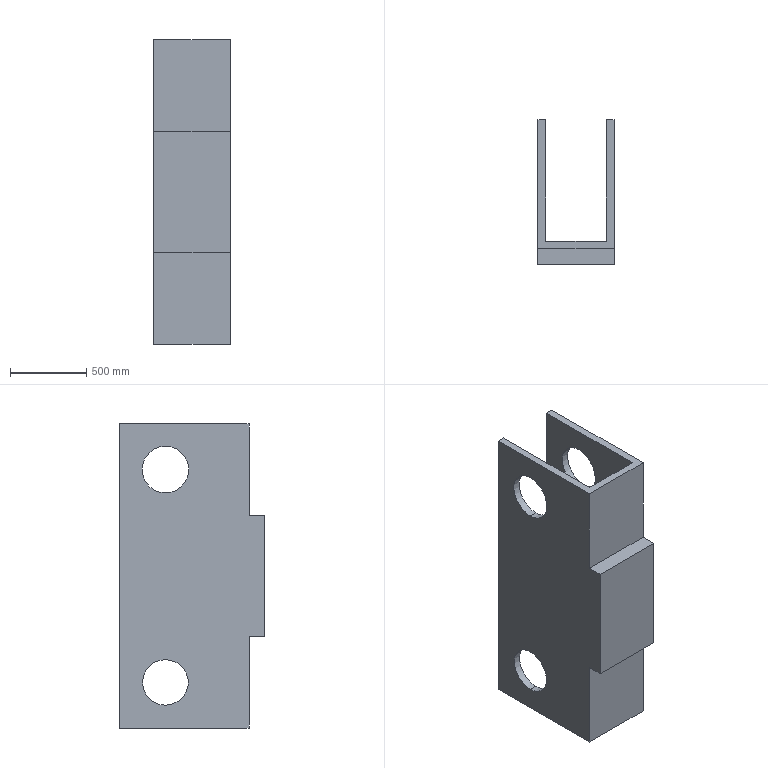Component | SolidWorks | LiftingAndOperatingMechanism-1_Part16-1 | 1 solid | 26 faces | box 500 x 950 x 2000 mm | volume 207505906 mm3 | plane 18 | cylinder 8 | commonest cylinder face diameters 300 x4 307.481 x4
build123d program:
from build123d import *

# Parameters (mm, degrees)
BOSS_EXTRUDE1_DEPTH = 250
SHELL1_T            = -50
SKETCH2_R           = 150
SKETCH2_R_2         = 153.74
CUT_EXTRUDE1_DEPTH  = 500


with BuildPart() as part:
    # Sketch1 → Boss-Extrude1 (new, symmetric)
    with BuildSketch(Plane(origin=(0, 0, 0), x_dir=(0, 0, -1), z_dir=(1, 0, 0))):
        Polygon((400, 425), (1000, 425), (1000, -425), (-1000, -425), (-1000, 425), (-400, 425), (-400, 525), (400, 525), align=None)
    extrude(amount=BOSS_EXTRUDE1_DEPTH, both=True)

    # Shell1
    shell1_openings = [part.faces().sort_by_distance(p)[0] for p in [
        (0, 0, 1000),
        (0, -425, 0),
        (0, 0, -1000),
    ]]
    offset(amount=SHELL1_T, openings=shell1_openings, kind=Kind.INTERSECTION)

    # Sketch2 → Cut-Extrude1 (cut)
    with BuildSketch(Plane(origin=(250, 0, 0), x_dir=(0, 0, -1), z_dir=(1, 0, 0))):
        with Locations((700, -125)):
            Circle(SKETCH2_R)
        with Locations((-700, -125)):
            Circle(SKETCH2_R_2)
    extrude(amount=-CUT_EXTRUDE1_DEPTH, mode=Mode.SUBTRACT)


solid = part.part

# Placed as in the assembly
solid = solid.moved(Location((2876.037, 13443.918, 4782.152), (0, 0, 180)))
STEP:
#1=COLOUR_RGB('',0.7922,0.8196,0.9333);
#2=FILL_AREA_STYLE_COLOUR('',#1);
#3=FILL_AREA_STYLE('',(#2));
#4=SURFACE_STYLE_FILL_AREA(#3);
#5=SURFACE_SIDE_STYLE('',(#4));
#6=SURFACE_STYLE_USAGE(.BOTH.,#5);
#7=PRESENTATION_STYLE_ASSIGNMENT((#6));
#8=CARTESIAN_POINT('',(105.356,534.209,154.809));
#9=VERTEX_POINT('',#8);
#10=CARTESIAN_POINT('',(105.356,534.209,166.62));
#11=VERTEX_POINT('',#10);
#12=CARTESIAN_POINT('',(105.356,534.209,160.715));
#13=DIRECTION('',(1.,0.,-0.0000002));
#14=DIRECTION('',(0.0000002,0.,1.));
#15=AXIS2_PLACEMENT_3D('',#12,#13,#14);
#16=CIRCLE('',#15,5.906);
#17=EDGE_CURVE('',#9,#11,#16,.T.);
#18=ORIENTED_EDGE('',*,*,#17,.T.);
#19=CARTESIAN_POINT('',(103.387,534.209,166.62));
#20=VERTEX_POINT('',#19);
#21=CARTESIAN_POINT('',(123.072,534.209,166.62));
#22=DIRECTION('',(-1.,-0.,0.0000002));
#23=VECTOR('',#22,39.37);
#24=LINE('',#21,#23);
#25=EDGE_CURVE('',#11,#20,#24,.T.);
#26=ORIENTED_EDGE('',*,*,#25,.T.);
#27=CARTESIAN_POINT('',(103.387,534.209,154.809));
#28=VERTEX_POINT('',#27);
#29=CARTESIAN_POINT('',(103.387,534.209,160.715));
#30=DIRECTION('',(-1.,-0.,0.0000002));
#31=DIRECTION('',(-0.0000002,0.,-1.));
#32=AXIS2_PLACEMENT_3D('',#29,#30,#31);
#33=CIRCLE('',#32,5.906);
#34=EDGE_CURVE('',#20,#28,#33,.T.);
#35=ORIENTED_EDGE('',*,*,#34,.T.);
#36=CARTESIAN_POINT('',(123.072,534.209,154.809));
#37=DIRECTION('',(-1.,-0.,0.0000002));
#38=VECTOR('',#37,39.37);
#39=LINE('',#36,#38);
#40=EDGE_CURVE('',#9,#28,#39,.T.);
#41=ORIENTED_EDGE('',*,*,#40,.F.);
#42=EDGE_LOOP('',(#18,#26,#35,#41));
#43=FACE_OUTER_BOUND('',#42,.T.);
#44=CARTESIAN_POINT('',(123.072,534.209,160.715));
#45=DIRECTION('',(-1.,-0.,0.0000002));
#46=DIRECTION('',(-0.0000002,0.,-1.));
#47=AXIS2_PLACEMENT_3D('',#44,#45,#46);
#48=CYLINDRICAL_SURFACE('',#47,5.906);
#49=ADVANCED_FACE('',(#43),#48,.F.);
#50=CARTESIAN_POINT('',(105.356,534.209,209.78));
#51=VERTEX_POINT('',#50);
#52=CARTESIAN_POINT('',(105.356,534.209,221.886));
#53=VERTEX_POINT('',#52);
#54=CARTESIAN_POINT('',(105.356,534.209,215.833));
#55=DIRECTION('',(1.,0.,-0.0000002));
#56=DIRECTION('',(0.0000002,0.,1.));
#57=AXIS2_PLACEMENT_3D('',#54,#55,#56);
#58=CIRCLE('',#57,6.053);
#59=EDGE_CURVE('',#51,#53,#58,.T.);
#60=ORIENTED_EDGE('',*,*,#59,.T.);
#61=CARTESIAN_POINT('',(103.387,534.209,221.886));
#62=VERTEX_POINT('',#61);
#63=CARTESIAN_POINT('',(123.072,534.209,221.886));
#64=DIRECTION('',(-1.,-0.,0.0000002));
#65=VECTOR('',#64,39.37);
#66=LINE('',#63,#65);
#67=EDGE_CURVE('',#53,#62,#66,.T.);
#68=ORIENTED_EDGE('',*,*,#67,.T.);
#69=CARTESIAN_POINT('',(103.387,534.209,209.78));
#70=VERTEX_POINT('',#69);
#71=CARTESIAN_POINT('',(103.387,534.209,215.833));
#72=DIRECTION('',(-1.,-0.,0.0000002));
#73=DIRECTION('',(-0.0000002,0.,-1.));
#74=AXIS2_PLACEMENT_3D('',#71,#72,#73);
#75=CIRCLE('',#74,6.053);
#76=EDGE_CURVE('',#62,#70,#75,.T.);
#77=ORIENTED_EDGE('',*,*,#76,.T.);
#78=CARTESIAN_POINT('',(123.072,534.209,209.78));
#79=DIRECTION('',(-1.,-0.,0.0000002));
#80=VECTOR('',#79,39.37);
#81=LINE('',#78,#80);
#82=EDGE_CURVE('',#51,#70,#81,.T.);
#83=ORIENTED_EDGE('',*,*,#82,.F.);
#84=EDGE_LOOP('',(#60,#68,#77,#83));
#85=FACE_OUTER_BOUND('',#84,.T.);
#86=CARTESIAN_POINT('',(123.072,534.209,215.833));
#87=DIRECTION('',(-1.,-0.,0.0000002));
#88=DIRECTION('',(-0.0000002,0.,-1.));
#89=AXIS2_PLACEMENT_3D('',#86,#87,#88);
#90=CYLINDRICAL_SURFACE('',#89,6.053);
#91=ADVANCED_FACE('',(#85),#90,.F.);
#92=CARTESIAN_POINT('',(123.072,534.209,166.62));
#93=VERTEX_POINT('',#92);
#94=CARTESIAN_POINT('',(123.072,534.209,154.809));
#95=VERTEX_POINT('',#94);
#96=CARTESIAN_POINT('',(123.072,534.209,160.715));
#97=DIRECTION('',(-1.,-0.,0.0000002));
#98=DIRECTION('',(-0.0000002,0.,-1.));
#99=AXIS2_PLACEMENT_3D('',#96,#97,#98);
#100=CIRCLE('',#99,5.906);
#101=EDGE_CURVE('',#93,#95,#100,.T.);
#102=ORIENTED_EDGE('',*,*,#101,.F.);
#103=CARTESIAN_POINT('',(121.104,534.209,166.62));
#104=VERTEX_POINT('',#103);
#105=CARTESIAN_POINT('',(123.072,534.209,166.62));
#106=DIRECTION('',(-1.,-0.,0.0000002));
#107=VECTOR('',#106,39.37);
#108=LINE('',#105,#107);
#109=EDGE_CURVE('',#93,#104,#108,.T.);
#110=ORIENTED_EDGE('',*,*,#109,.T.);
#111=CARTESIAN_POINT('',(121.104,534.209,154.809));
#112=VERTEX_POINT('',#111);
#113=CARTESIAN_POINT('',(121.104,534.209,160.715));
#114=DIRECTION('',(1.,0.,-0.0000002));
#115=DIRECTION('',(0.0000002,0.,1.));
#116=AXIS2_PLACEMENT_3D('',#113,#114,#115);
#117=CIRCLE('',#116,5.906);
#118=EDGE_CURVE('',#112,#104,#117,.T.);
#119=ORIENTED_EDGE('',*,*,#118,.F.);
#120=CARTESIAN_POINT('',(123.072,534.209,154.809));
#121=DIRECTION('',(-1.,-0.,0.0000002));
#122=VECTOR('',#121,39.37);
#123=LINE('',#120,#122);
#124=EDGE_CURVE('',#95,#112,#123,.T.);
#125=ORIENTED_EDGE('',*,*,#124,.F.);
#126=EDGE_LOOP('',(#102,#110,#119,#125));
#127=FACE_OUTER_BOUND('',#126,.T.);
#128=CARTESIAN_POINT('',(123.072,534.209,160.715));
#129=DIRECTION('',(-1.,-0.,0.0000002));
#130=DIRECTION('',(-0.0000002,0.,-1.));
#131=AXIS2_PLACEMENT_3D('',#128,#129,#130);
#132=CYLINDRICAL_SURFACE('',#131,5.906);
#133=ADVANCED_FACE('',(#127),#132,.F.);
#134=CARTESIAN_POINT('',(123.072,534.209,221.886));
#135=VERTEX_POINT('',#134);
#136=CARTESIAN_POINT('',(123.072,534.209,209.78));
#137=VERTEX_POINT('',#136);
#138=CARTESIAN_POINT('',(123.072,534.209,215.833));
#139=DIRECTION('',(-1.,-0.,0.0000002));
#140=DIRECTION('',(-0.0000002,0.,-1.));
#141=AXIS2_PLACEMENT_3D('',#138,#139,#140);
#142=CIRCLE('',#141,6.053);
#143=EDGE_CURVE('',#135,#137,#142,.T.);
#144=ORIENTED_EDGE('',*,*,#143,.F.);
#145=CARTESIAN_POINT('',(121.104,534.209,221.886));
#146=VERTEX_POINT('',#145);
#147=CARTESIAN_POINT('',(123.072,534.209,221.886));
#148=DIRECTION('',(-1.,-0.,0.0000002));
#149=VECTOR('',#148,39.37);
#150=LINE('',#147,#149);
#151=EDGE_CURVE('',#135,#146,#150,.T.);
#152=ORIENTED_EDGE('',*,*,#151,.T.);
#153=CARTESIAN_POINT('',(121.104,534.209,209.78));
#154=VERTEX_POINT('',#153);
#155=CARTESIAN_POINT('',(121.104,534.209,215.833));
#156=DIRECTION('',(1.,0.,-0.0000002));
#157=DIRECTION('',(0.0000002,0.,1.));
#158=AXIS2_PLACEMENT_3D('',#155,#156,#157);
#159=CIRCLE('',#158,6.053);
#160=EDGE_CURVE('',#154,#146,#159,.T.);
#161=ORIENTED_EDGE('',*,*,#160,.F.);
#162=CARTESIAN_POINT('',(123.072,534.209,209.78));
#163=DIRECTION('',(-1.,-0.,0.0000002));
#164=VECTOR('',#163,39.37);
#165=LINE('',#162,#164);
#166=EDGE_CURVE('',#137,#154,#165,.T.);
#167=ORIENTED_EDGE('',*,*,#166,.F.);
#168=EDGE_LOOP('',(#144,#152,#161,#167));
#169=FACE_OUTER_BOUND('',#168,.T.);
#170=CARTESIAN_POINT('',(123.072,534.209,215.833));
#171=DIRECTION('',(-1.,-0.,0.0000002));
#172=DIRECTION('',(-0.0000002,0.,-1.));
#173=AXIS2_PLACEMENT_3D('',#170,#171,#172);
#174=CYLINDRICAL_SURFACE('',#173,6.053);
#175=ADVANCED_FACE('',(#169),#174,.F.);
#176=CARTESIAN_POINT('',(121.104,546.02,148.904));
#177=VERTEX_POINT('',#176);
#178=CARTESIAN_POINT('',(121.104,514.524,148.904));
#179=VERTEX_POINT('',#178);
#180=CARTESIAN_POINT('',(121.104,529.288,148.904));
#181=DIRECTION('',(0.,-1.,-0.));
#182=VECTOR('',#181,39.37);
#183=LINE('',#180,#182);
#184=EDGE_CURVE('',#177,#179,#183,.T.);
#185=ORIENTED_EDGE('',*,*,#184,.F.);
#186=CARTESIAN_POINT('',(123.072,546.02,148.904));
#187=VERTEX_POINT('',#186);
#188=CARTESIAN_POINT('',(103.387,546.02,148.904));
#189=DIRECTION('',(1.,0.,-0.0000002));
#190=VECTOR('',#189,39.37);
#191=LINE('',#188,#190);
#192=EDGE_CURVE('',#177,#187,#191,.T.);
#193=ORIENTED_EDGE('',*,*,#192,.T.);
#194=CARTESIAN_POINT('',(123.072,512.556,148.904));
#195=VERTEX_POINT('',#194);
#196=CARTESIAN_POINT('',(123.072,546.02,148.904));
#197=DIRECTION('',(0.,-1.,-0.));
#198=VECTOR('',#197,39.37);
#199=LINE('',#196,#198);
#200=EDGE_CURVE('',#187,#195,#199,.T.);
#201=ORIENTED_EDGE('',*,*,#200,.T.);
#202=CARTESIAN_POINT('',(103.387,512.556,148.904));
#203=VERTEX_POINT('',#202);
#204=CARTESIAN_POINT('',(103.387,512.556,148.904));
#205=DIRECTION('',(1.,0.,-0.0000002));
#206=VECTOR('',#205,39.37);
#207=LINE('',#204,#206);
#208=EDGE_CURVE('',#203,#195,#207,.T.);
#209=ORIENTED_EDGE('',*,*,#208,.F.);
#210=CARTESIAN_POINT('',(103.387,546.02,148.904));
#211=VERTEX_POINT('',#210);
#212=CARTESIAN_POINT('',(103.387,546.02,148.904));
#213=DIRECTION('',(0.,-1.,-0.));
#214=VECTOR('',#213,39.37);
#215=LINE('',#212,#214);
#216=EDGE_CURVE('',#211,#203,#215,.T.);
#217=ORIENTED_EDGE('',*,*,#216,.F.);
#218=CARTESIAN_POINT('',(105.356,546.02,148.904));
#219=VERTEX_POINT('',#218);
#220=CARTESIAN_POINT('',(103.387,546.02,148.904));
#221=DIRECTION('',(1.,0.,-0.0000002));
#222=VECTOR('',#221,39.37);
#223=LINE('',#220,#222);
#224=EDGE_CURVE('',#211,#219,#223,.T.);
#225=ORIENTED_EDGE('',*,*,#224,.T.);
#226=CARTESIAN_POINT('',(105.356,514.524,148.904));
#227=VERTEX_POINT('',#226);
#228=CARTESIAN_POINT('',(105.356,529.288,148.904));
#229=DIRECTION('',(0.,-1.,-0.));
#230=VECTOR('',#229,39.37);
#231=LINE('',#228,#230);
#232=EDGE_CURVE('',#219,#227,#231,.T.);
#233=ORIENTED_EDGE('',*,*,#232,.T.);
#234=CARTESIAN_POINT('',(103.387,514.524,148.904));
#235=DIRECTION('',(1.,0.,-0.0000002));
#236=VECTOR('',#235,39.37);
#237=LINE('',#234,#236);
#238=EDGE_CURVE('',#227,#179,#237,.T.);
#239=ORIENTED_EDGE('',*,*,#238,.T.);
#240=EDGE_LOOP('',(#185,#193,#201,#209,#217,#225,#233,#239));
#241=FACE_OUTER_BOUND('',#240,.T.);
#242=CARTESIAN_POINT('',(103.387,546.02,148.904));
#243=DIRECTION('',(0.0000002,-0.,1.));
#244=DIRECTION('',(-1.,-0.,0.0000002));
#245=AXIS2_PLACEMENT_3D('',#242,#243,#244);
#246=PLANE('',#245);
#247=ADVANCED_FACE('',(#241),#246,.F.);
#248=CARTESIAN_POINT('',(121.104,514.524,227.644));
#249=VERTEX_POINT('',#248);
#250=CARTESIAN_POINT('',(121.104,546.02,227.644));
#251=VERTEX_POINT('',#250);
#252=CARTESIAN_POINT('',(121.104,529.288,227.644));
#253=DIRECTION('',(-0.,1.,0.));
#254=VECTOR('',#253,39.37);
#255=LINE('',#252,#254);
#256=EDGE_CURVE('',#249,#251,#255,.T.);
#257=ORIENTED_EDGE('',*,*,#256,.F.);
#258=CARTESIAN_POINT('',(105.356,514.524,227.644));
#259=VERTEX_POINT('',#258);
#260=CARTESIAN_POINT('',(103.387,514.524,227.644));
#261=DIRECTION('',(1.,0.,-0.0000002));
#262=VECTOR('',#261,39.37);
#263=LINE('',#260,#262);
#264=EDGE_CURVE('',#259,#249,#263,.T.);
#265=ORIENTED_EDGE('',*,*,#264,.F.);
#266=CARTESIAN_POINT('',(105.356,546.02,227.644));
#267=VERTEX_POINT('',#266);
#268=CARTESIAN_POINT('',(105.356,529.288,227.644));
#269=DIRECTION('',(-0.,1.,0.));
#270=VECTOR('',#269,39.37);
#271=LINE('',#268,#270);
#272=EDGE_CURVE('',#259,#267,#271,.T.);
#273=ORIENTED_EDGE('',*,*,#272,.T.);
#274=CARTESIAN_POINT('',(103.387,546.02,227.644));
#275=VERTEX_POINT('',#274);
#276=CARTESIAN_POINT('',(103.387,546.02,227.644));
#277=DIRECTION('',(1.,0.,-0.0000002));
#278=VECTOR('',#277,39.37);
#279=LINE('',#276,#278);
#280=EDGE_CURVE('',#275,#267,#279,.T.);
#281=ORIENTED_EDGE('',*,*,#280,.F.);
#282=CARTESIAN_POINT('',(103.387,512.556,227.644));
#283=VERTEX_POINT('',#282);
#284=CARTESIAN_POINT('',(103.387,546.02,227.644));
#285=DIRECTION('',(-0.,1.,0.));
#286=VECTOR('',#285,39.37);
#287=LINE('',#284,#286);
#288=EDGE_CURVE('',#283,#275,#287,.T.);
#289=ORIENTED_EDGE('',*,*,#288,.F.);
#290=CARTESIAN_POINT('',(123.072,512.556,227.644));
#291=VERTEX_POINT('',#290);
#292=CARTESIAN_POINT('',(103.387,512.556,227.644));
#293=DIRECTION('',(1.,0.,-0.0000002));
#294=VECTOR('',#293,39.37);
#295=LINE('',#292,#294);
#296=EDGE_CURVE('',#283,#291,#295,.T.);
#297=ORIENTED_EDGE('',*,*,#296,.T.);
#298=CARTESIAN_POINT('',(123.072,546.02,227.644));
#299=VERTEX_POINT('',#298);
#300=CARTESIAN_POINT('',(123.072,546.02,227.644));
#301=DIRECTION('',(-0.,1.,0.));
#302=VECTOR('',#301,39.37);
#303=LINE('',#300,#302);
#304=EDGE_CURVE('',#291,#299,#303,.T.);
#305=ORIENTED_EDGE('',*,*,#304,.T.);
#306=CARTESIAN_POINT('',(103.387,546.02,227.644));
#307=DIRECTION('',(1.,0.,-0.0000002));
#308=VECTOR('',#307,39.37);
#309=LINE('',#306,#308);
#310=EDGE_CURVE('',#251,#299,#309,.T.);
#311=ORIENTED_EDGE('',*,*,#310,.F.);
#312=EDGE_LOOP('',(#257,#265,#273,#281,#289,#297,#305,#311));
#313=FACE_OUTER_BOUND('',#312,.T.);
#314=CARTESIAN_POINT('',(103.387,546.02,227.644));
#315=DIRECTION('',(-0.0000002,0.,-1.));
#316=DIRECTION('',(1.,0.,-0.0000002));
#317=AXIS2_PLACEMENT_3D('',#314,#315,#316);
#318=PLANE('',#317);
#319=ADVANCED_FACE('',(#313),#318,.F.);
#320=CARTESIAN_POINT('',(121.104,546.02,188.274));
#321=DIRECTION('',(-0.0000002,0.,-1.));
#322=VECTOR('',#321,39.37);
#323=LINE('',#320,#322);
#324=EDGE_CURVE('',#251,#177,#323,.T.);
#325=ORIENTED_EDGE('',*,*,#324,.F.);
#326=ORIENTED_EDGE('',*,*,#310,.T.);
#327=CARTESIAN_POINT('',(123.072,546.02,227.644));
#328=DIRECTION('',(-0.0000002,0.,-1.));
#329=VECTOR('',#328,39.37);
#330=LINE('',#327,#329);
#331=EDGE_CURVE('',#299,#187,#330,.T.);
#332=ORIENTED_EDGE('',*,*,#331,.T.);
#333=ORIENTED_EDGE('',*,*,#192,.F.);
#334=EDGE_LOOP('',(#325,#326,#332,#333));
#335=FACE_OUTER_BOUND('',#334,.T.);
#336=CARTESIAN_POINT('',(103.387,546.02,227.644));
#337=DIRECTION('',(0.,-1.,-0.));
#338=DIRECTION('',(0.0000002,-0.,1.));
#339=AXIS2_PLACEMENT_3D('',#336,#337,#338);
#340=PLANE('',#339);
#341=ADVANCED_FACE('',(#335),#340,.F.);
#342=CARTESIAN_POINT('',(123.072,512.556,172.526));
#343=VERTEX_POINT('',#342);
#344=CARTESIAN_POINT('',(123.072,512.556,172.526));
#345=DIRECTION('',(0.0000002,-0.,1.));
#346=VECTOR('',#345,39.37);
#347=LINE('',#344,#346);
#348=EDGE_CURVE('',#195,#343,#347,.T.);
#349=ORIENTED_EDGE('',*,*,#348,.T.);
#350=CARTESIAN_POINT('',(103.387,512.556,172.526));
#351=VERTEX_POINT('',#350);
#352=CARTESIAN_POINT('',(103.387,512.556,172.526));
#353=DIRECTION('',(1.,0.,-0.0000002));
#354=VECTOR('',#353,39.37);
#355=LINE('',#352,#354);
#356=EDGE_CURVE('',#351,#343,#355,.T.);
#357=ORIENTED_EDGE('',*,*,#356,.F.);
#358=CARTESIAN_POINT('',(103.387,512.556,172.526));
#359=DIRECTION('',(0.0000002,-0.,1.));
#360=VECTOR('',#359,39.37);
#361=LINE('',#358,#360);
#362=EDGE_CURVE('',#203,#351,#361,.T.);
#363=ORIENTED_EDGE('',*,*,#362,.F.);
#364=ORIENTED_EDGE('',*,*,#208,.T.);
#365=EDGE_LOOP('',(#349,#357,#363,#364));
#366=FACE_OUTER_BOUND('',#365,.T.);
#367=CARTESIAN_POINT('',(103.387,512.556,172.526));
#368=DIRECTION('',(-0.,1.,0.));
#369=DIRECTION('',(-0.0000002,0.,-1.));
#370=AXIS2_PLACEMENT_3D('',#367,#368,#369);
#371=PLANE('',#370);
#372=ADVANCED_FACE('',(#366),#371,.F.);
#373=CARTESIAN_POINT('',(123.072,508.619,172.526));
#374=VERTEX_POINT('',#373);
#375=CARTESIAN_POINT('',(123.072,512.556,172.526));
#376=DIRECTION('',(0.,-1.,-0.));
#377=VECTOR('',#376,39.37);
#378=LINE('',#375,#377);
#379=EDGE_CURVE('',#343,#374,#378,.T.);
#380=ORIENTED_EDGE('',*,*,#379,.T.);
#381=CARTESIAN_POINT('',(103.387,508.619,172.526));
#382=VERTEX_POINT('',#381);
#383=CARTESIAN_POINT('',(103.387,508.619,172.526));
#384=DIRECTION('',(1.,0.,-0.0000002));
#385=VECTOR('',#384,39.37);
#386=LINE('',#383,#385);
#387=EDGE_CURVE('',#382,#374,#386,.T.);
#388=ORIENTED_EDGE('',*,*,#387,.F.);
#389=CARTESIAN_POINT('',(103.387,512.556,172.526));
#390=DIRECTION('',(0.,-1.,-0.));
#391=VECTOR('',#390,39.37);
#392=LINE('',#389,#391);
#393=EDGE_CURVE('',#351,#382,#392,.T.);
#394=ORIENTED_EDGE('',*,*,#393,.F.);
#395=ORIENTED_EDGE('',*,*,#356,.T.);
#396=EDGE_LOOP('',(#380,#388,#394,#395));
#397=FACE_OUTER_BOUND('',#396,.T.);
#398=CARTESIAN_POINT('',(103.387,512.556,172.526));
#399=DIRECTION('',(0.0000002,-0.,1.));
#400=DIRECTION('',(-1.,-0.,0.0000002));
#401=AXIS2_PLACEMENT_3D('',#398,#399,#400);
#402=PLANE('',#401);
#403=ADVANCED_FACE('',(#397),#402,.F.);
#404=CARTESIAN_POINT('',(123.072,508.619,204.022));
#405=VERTEX_POINT('',#404);
#406=CARTESIAN_POINT('',(123.072,508.619,204.022));
#407=DIRECTION('',(0.0000002,-0.,1.));
#408=VECTOR('',#407,39.37);
#409=LINE('',#406,#408);
#410=EDGE_CURVE('',#374,#405,#409,.T.);
#411=ORIENTED_EDGE('',*,*,#410,.T.);
#412=CARTESIAN_POINT('',(103.387,508.619,204.022));
#413=VERTEX_POINT('',#412);
#414=CARTESIAN_POINT('',(103.387,508.619,204.022));
#415=DIRECTION('',(1.,0.,-0.0000002));
#416=VECTOR('',#415,39.37);
#417=LINE('',#414,#416);
#418=EDGE_CURVE('',#413,#405,#417,.T.);
#419=ORIENTED_EDGE('',*,*,#418,.F.);
#420=CARTESIAN_POINT('',(103.387,508.619,204.022));
#421=DIRECTION('',(0.0000002,-0.,1.));
#422=VECTOR('',#421,39.37);
#423=LINE('',#420,#422);
#424=EDGE_CURVE('',#382,#413,#423,.T.);
#425=ORIENTED_EDGE('',*,*,#424,.F.);
#426=ORIENTED_EDGE('',*,*,#387,.T.);
#427=EDGE_LOOP('',(#411,#419,#425,#426));
#428=FACE_OUTER_BOUND('',#427,.T.);
#429=CARTESIAN_POINT('',(103.387,508.619,204.022));
#430=DIRECTION('',(-0.,1.,0.));
#431=DIRECTION('',(-0.0000002,0.,-1.));
#432=AXIS2_PLACEMENT_3D('',#429,#430,#431);
#433=PLANE('',#432);
#434=ADVANCED_FACE('',(#428),#433,.F.);
#435=CARTESIAN_POINT('',(123.072,512.556,204.022));
#436=VERTEX_POINT('',#435);
#437=CARTESIAN_POINT('',(123.072,512.556,204.022));
#438=DIRECTION('',(-0.,1.,0.));
#439=VECTOR('',#438,39.37);
#440=LINE('',#437,#439);
#441=EDGE_CURVE('',#405,#436,#440,.T.);
#442=ORIENTED_EDGE('',*,*,#441,.T.);
#443=CARTESIAN_POINT('',(103.387,512.556,204.022));
#444=VERTEX_POINT('',#443);
#445=CARTESIAN_POINT('',(103.387,512.556,204.022));
#446=DIRECTION('',(1.,0.,-0.0000002));
#447=VECTOR('',#446,39.37);
#448=LINE('',#445,#447);
#449=EDGE_CURVE('',#444,#436,#448,.T.);
#450=ORIENTED_EDGE('',*,*,#449,.F.);
#451=CARTESIAN_POINT('',(103.387,512.556,204.022));
#452=DIRECTION('',(-0.,1.,0.));
#453=VECTOR('',#452,39.37);
#454=LINE('',#451,#453);
#455=EDGE_CURVE('',#413,#444,#454,.T.);
#456=ORIENTED_EDGE('',*,*,#455,.F.);
#457=ORIENTED_EDGE('',*,*,#418,.T.);
#458=EDGE_LOOP('',(#442,#450,#456,#457));
#459=FACE_OUTER_BOUND('',#458,.T.);
#460=CARTESIAN_POINT('',(103.387,512.556,204.022));
#461=DIRECTION('',(-0.0000002,0.,-1.));
#462=DIRECTION('',(1.,0.,-0.0000002));
#463=AXIS2_PLACEMENT_3D('',#460,#461,#462);
#464=PLANE('',#463);
#465=ADVANCED_FACE('',(#459),#464,.F.);
#466=CARTESIAN_POINT('',(123.072,512.556,227.644));
#467=DIRECTION('',(0.0000002,-0.,1.));
#468=VECTOR('',#467,39.37);
#469=LINE('',#466,#468);
#470=EDGE_CURVE('',#436,#291,#469,.T.);
#471=ORIENTED_EDGE('',*,*,#470,.T.);
#472=ORIENTED_EDGE('',*,*,#296,.F.);
#473=CARTESIAN_POINT('',(103.387,512.556,227.644));
#474=DIRECTION('',(0.0000002,-0.,1.));
#475=VECTOR('',#474,39.37);
#476=LINE('',#473,#475);
#477=EDGE_CURVE('',#444,#283,#476,.T.);
#478=ORIENTED_EDGE('',*,*,#477,.F.);
#479=ORIENTED_EDGE('',*,*,#449,.T.);
#480=EDGE_LOOP('',(#471,#472,#478,#479));
#481=FACE_OUTER_BOUND('',#480,.T.);
#482=CARTESIAN_POINT('',(103.387,512.556,227.644));
#483=DIRECTION('',(-0.,1.,0.));
#484=DIRECTION('',(-0.0000002,0.,-1.));
#485=AXIS2_PLACEMENT_3D('',#482,#483,#484);
#486=PLANE('',#485);
#487=ADVANCED_FACE('',(#481),#486,.F.);
#488=ORIENTED_EDGE('',*,*,#280,.T.);
#489=CARTESIAN_POINT('',(105.356,546.02,188.274));
#490=DIRECTION('',(-0.0000002,0.,-1.));
#491=VECTOR('',#490,39.37);
#492=LINE('',#489,#491);
#493=EDGE_CURVE('',#267,#219,#492,.T.);
#494=ORIENTED_EDGE('',*,*,#493,.T.);
#495=ORIENTED_EDGE('',*,*,#224,.F.);
#496=CARTESIAN_POINT('',(103.387,546.02,227.644));
#497=DIRECTION('',(-0.0000002,0.,-1.));
#498=VECTOR('',#497,39.37);
#499=LINE('',#496,#498);
#500=EDGE_CURVE('',#275,#211,#499,.T.);
#501=ORIENTED_EDGE('',*,*,#500,.F.);
#502=EDGE_LOOP('',(#488,#494,#495,#501));
#503=FACE_OUTER_BOUND('',#502,.T.);
#504=CARTESIAN_POINT('',(103.387,546.02,227.644));
#505=DIRECTION('',(0.,-1.,-0.));
#506=DIRECTION('',(0.0000002,-0.,1.));
#507=AXIS2_PLACEMENT_3D('',#504,#505,#506);
#508=PLANE('',#507);
#509=ADVANCED_FACE('',(#503),#508,.F.);
#510=CARTESIAN_POINT('',(103.387,534.209,160.715));
#511=DIRECTION('',(-1.,-0.,0.0000002));
#512=DIRECTION('',(-0.0000002,0.,-1.));
#513=AXIS2_PLACEMENT_3D('',#510,#511,#512);
#514=CIRCLE('',#513,5.906);
#515=EDGE_CURVE('',#28,#20,#514,.T.);
#516=ORIENTED_EDGE('',*,*,#515,.F.);
#517=ORIENTED_EDGE('',*,*,#34,.F.);
#518=EDGE_LOOP('',(#516,#517));
#519=FACE_BOUND('',#518,.T.);
#520=CARTESIAN_POINT('',(103.387,534.209,215.833));
#521=DIRECTION('',(-1.,-0.,0.0000002));
#522=DIRECTION('',(-0.0000002,0.,-1.));
#523=AXIS2_PLACEMENT_3D('',#520,#521,#522);
#524=CIRCLE('',#523,6.053);
#525=EDGE_CURVE('',#70,#62,#524,.T.);
#526=ORIENTED_EDGE('',*,*,#525,.F.);
#527=ORIENTED_EDGE('',*,*,#76,.F.);
#528=EDGE_LOOP('',(#526,#527));
#529=FACE_BOUND('',#528,.T.);
#530=ORIENTED_EDGE('',*,*,#216,.T.);
#531=ORIENTED_EDGE('',*,*,#362,.T.);
#532=ORIENTED_EDGE('',*,*,#393,.T.);
#533=ORIENTED_EDGE('',*,*,#424,.T.);
#534=ORIENTED_EDGE('',*,*,#455,.T.);
#535=ORIENTED_EDGE('',*,*,#477,.T.);
#536=ORIENTED_EDGE('',*,*,#288,.T.);
#537=ORIENTED_EDGE('',*,*,#500,.T.);
#538=EDGE_LOOP('',(#530,#531,#532,#533,#534,#535,#536,#537));
#539=FACE_OUTER_BOUND('',#538,.T.);
#540=CARTESIAN_POINT('',(103.387,529.288,188.274));
#541=DIRECTION('',(1.,0.,-0.0000002));
#542=DIRECTION('',(0.0000002,-0.,1.));
#543=AXIS2_PLACEMENT_3D('',#540,#541,#542);
#544=PLANE('',#543);
#545=ADVANCED_FACE('',(#519,#529,#539),#544,.F.);
#546=CARTESIAN_POINT('',(123.072,534.209,160.715));
#547=DIRECTION('',(-1.,-0.,0.0000002));
#548=DIRECTION('',(-0.0000002,0.,-1.));
#549=AXIS2_PLACEMENT_3D('',#546,#547,#548);
#550=CIRCLE('',#549,5.906);
#551=EDGE_CURVE('',#95,#93,#550,.T.);
#552=ORIENTED_EDGE('',*,*,#551,.T.);
#553=ORIENTED_EDGE('',*,*,#101,.T.);
#554=EDGE_LOOP('',(#552,#553));
#555=FACE_BOUND('',#554,.T.);
#556=CARTESIAN_POINT('',(123.072,534.209,215.833));
#557=DIRECTION('',(-1.,-0.,0.0000002));
#558=DIRECTION('',(-0.0000002,0.,-1.));
#559=AXIS2_PLACEMENT_3D('',#556,#557,#558);
#560=CIRCLE('',#559,6.053);
#561=EDGE_CURVE('',#137,#135,#560,.T.);
#562=ORIENTED_EDGE('',*,*,#561,.T.);
#563=ORIENTED_EDGE('',*,*,#143,.T.);
#564=EDGE_LOOP('',(#562,#563));
#565=FACE_BOUND('',#564,.T.);
#566=ORIENTED_EDGE('',*,*,#200,.F.);
#567=ORIENTED_EDGE('',*,*,#331,.F.);
#568=ORIENTED_EDGE('',*,*,#304,.F.);
#569=ORIENTED_EDGE('',*,*,#470,.F.);
#570=ORIENTED_EDGE('',*,*,#441,.F.);
#571=ORIENTED_EDGE('',*,*,#410,.F.);
#572=ORIENTED_EDGE('',*,*,#379,.F.);
#573=ORIENTED_EDGE('',*,*,#348,.F.);
#574=EDGE_LOOP('',(#566,#567,#568,#569,#570,#571,#572,#573));
#575=FACE_OUTER_BOUND('',#574,.T.);
#576=CARTESIAN_POINT('',(123.072,529.288,188.274));
#577=DIRECTION('',(1.,0.,-0.0000002));
#578=DIRECTION('',(0.0000002,-0.,1.));
#579=AXIS2_PLACEMENT_3D('',#576,#577,#578);
#580=PLANE('',#579);
#581=ADVANCED_FACE('',(#555,#565,#575),#580,.T.);
#582=CARTESIAN_POINT('',(121.104,514.524,174.494));
#583=VERTEX_POINT('',#582);
#584=CARTESIAN_POINT('',(121.104,514.524,188.274));
#585=DIRECTION('',(0.0000002,-0.,1.));
#586=VECTOR('',#585,39.37);
#587=LINE('',#584,#586);
#588=EDGE_CURVE('',#179,#583,#587,.T.);
#589=ORIENTED_EDGE('',*,*,#588,.F.);
#590=ORIENTED_EDGE('',*,*,#238,.F.);
#591=CARTESIAN_POINT('',(105.356,514.524,174.494));
#592=VERTEX_POINT('',#591);
#593=CARTESIAN_POINT('',(105.356,514.524,188.274));
#594=DIRECTION('',(0.0000002,-0.,1.));
#595=VECTOR('',#594,39.37);
#596=LINE('',#593,#595);
#597=EDGE_CURVE('',#227,#592,#596,.T.);
#598=ORIENTED_EDGE('',*,*,#597,.T.);
#599=CARTESIAN_POINT('',(103.387,514.524,174.494));
#600=DIRECTION('',(1.,0.,-0.0000002));
#601=VECTOR('',#600,39.37);
#602=LINE('',#599,#601);
#603=EDGE_CURVE('',#592,#583,#602,.T.);
#604=ORIENTED_EDGE('',*,*,#603,.T.);
#605=EDGE_LOOP('',(#589,#590,#598,#604));
#606=FACE_OUTER_BOUND('',#605,.T.);
#607=CARTESIAN_POINT('',(103.387,514.524,172.526));
#608=DIRECTION('',(-0.,1.,0.));
#609=DIRECTION('',(-0.0000002,0.,-1.));
#610=AXIS2_PLACEMENT_3D('',#607,#608,#609);
#611=PLANE('',#610);
#612=ADVANCED_FACE('',(#606),#611,.T.);
#613=CARTESIAN_POINT('',(121.104,510.587,174.494));
#614=VERTEX_POINT('',#613);
#615=CARTESIAN_POINT('',(121.104,529.288,174.494));
#616=DIRECTION('',(0.,-1.,-0.));
#617=VECTOR('',#616,39.37);
#618=LINE('',#615,#617);
#619=EDGE_CURVE('',#583,#614,#618,.T.);
#620=ORIENTED_EDGE('',*,*,#619,.F.);
#621=ORIENTED_EDGE('',*,*,#603,.F.);
#622=CARTESIAN_POINT('',(105.356,510.587,174.494));
#623=VERTEX_POINT('',#622);
#624=CARTESIAN_POINT('',(105.356,529.288,174.494));
#625=DIRECTION('',(0.,-1.,-0.));
#626=VECTOR('',#625,39.37);
#627=LINE('',#624,#626);
#628=EDGE_CURVE('',#592,#623,#627,.T.);
#629=ORIENTED_EDGE('',*,*,#628,.T.);
#630=CARTESIAN_POINT('',(103.387,510.587,174.494));
#631=DIRECTION('',(1.,0.,-0.0000002));
#632=VECTOR('',#631,39.37);
#633=LINE('',#630,#632);
#634=EDGE_CURVE('',#623,#614,#633,.T.);
#635=ORIENTED_EDGE('',*,*,#634,.T.);
#636=EDGE_LOOP('',(#620,#621,#629,#635));
#637=FACE_OUTER_BOUND('',#636,.T.);
#638=CARTESIAN_POINT('',(103.387,512.556,174.494));
#639=DIRECTION('',(0.0000002,-0.,1.));
#640=DIRECTION('',(-1.,-0.,0.0000002));
#641=AXIS2_PLACEMENT_3D('',#638,#639,#640);
#642=PLANE('',#641);
#643=ADVANCED_FACE('',(#637),#642,.T.);
#644=CARTESIAN_POINT('',(121.104,510.587,202.053));
#645=VERTEX_POINT('',#644);
#646=CARTESIAN_POINT('',(121.104,510.587,188.274));
#647=DIRECTION('',(0.0000002,-0.,1.));
#648=VECTOR('',#647,39.37);
#649=LINE('',#646,#648);
#650=EDGE_CURVE('',#614,#645,#649,.T.);
#651=ORIENTED_EDGE('',*,*,#650,.F.);
#652=ORIENTED_EDGE('',*,*,#634,.F.);
#653=CARTESIAN_POINT('',(105.356,510.587,202.053));
#654=VERTEX_POINT('',#653);
#655=CARTESIAN_POINT('',(105.356,510.587,188.274));
#656=DIRECTION('',(0.0000002,-0.,1.));
#657=VECTOR('',#656,39.37);
#658=LINE('',#655,#657);
#659=EDGE_CURVE('',#623,#654,#658,.T.);
#660=ORIENTED_EDGE('',*,*,#659,.T.);
#661=CARTESIAN_POINT('',(103.387,510.587,202.053));
#662=DIRECTION('',(1.,0.,-0.0000002));
#663=VECTOR('',#662,39.37);
#664=LINE('',#661,#663);
#665=EDGE_CURVE('',#654,#645,#664,.T.);
#666=ORIENTED_EDGE('',*,*,#665,.T.);
#667=EDGE_LOOP('',(#651,#652,#660,#666));
#668=FACE_OUTER_BOUND('',#667,.T.);
#669=CARTESIAN_POINT('',(103.387,510.587,204.022));
#670=DIRECTION('',(-0.,1.,0.));
#671=DIRECTION('',(-0.0000002,0.,-1.));
#672=AXIS2_PLACEMENT_3D('',#669,#670,#671);
#673=PLANE('',#672);
#674=ADVANCED_FACE('',(#668),#673,.T.);
#675=CARTESIAN_POINT('',(121.104,514.524,202.053));
#676=VERTEX_POINT('',#675);
#677=CARTESIAN_POINT('',(121.104,529.288,202.053));
#678=DIRECTION('',(-0.,1.,0.));
#679=VECTOR('',#678,39.37);
#680=LINE('',#677,#679);
#681=EDGE_CURVE('',#645,#676,#680,.T.);
#682=ORIENTED_EDGE('',*,*,#681,.F.);
#683=ORIENTED_EDGE('',*,*,#665,.F.);
#684=CARTESIAN_POINT('',(105.356,514.524,202.053));
#685=VERTEX_POINT('',#684);
#686=CARTESIAN_POINT('',(105.356,529.288,202.053));
#687=DIRECTION('',(-0.,1.,0.));
#688=VECTOR('',#687,39.37);
#689=LINE('',#686,#688);
#690=EDGE_CURVE('',#654,#685,#689,.T.);
#691=ORIENTED_EDGE('',*,*,#690,.T.);
#692=CARTESIAN_POINT('',(103.387,514.524,202.053));
#693=DIRECTION('',(1.,0.,-0.0000002));
#694=VECTOR('',#693,39.37);
#695=LINE('',#692,#694);
#696=EDGE_CURVE('',#685,#676,#695,.T.);
#697=ORIENTED_EDGE('',*,*,#696,.T.);
#698=EDGE_LOOP('',(#682,#683,#691,#697));
#699=FACE_OUTER_BOUND('',#698,.T.);
#700=CARTESIAN_POINT('',(103.387,512.556,202.053));
#701=DIRECTION('',(-0.0000002,0.,-1.));
#702=DIRECTION('',(1.,0.,-0.0000002));
#703=AXIS2_PLACEMENT_3D('',#700,#701,#702);
#704=PLANE('',#703);
#705=ADVANCED_FACE('',(#699),#704,.T.);
#706=CARTESIAN_POINT('',(121.104,514.524,188.274));
#707=DIRECTION('',(0.0000002,-0.,1.));
#708=VECTOR('',#707,39.37);
#709=LINE('',#706,#708);
#710=EDGE_CURVE('',#676,#249,#709,.T.);
#711=ORIENTED_EDGE('',*,*,#710,.F.);
#712=ORIENTED_EDGE('',*,*,#696,.F.);
#713=CARTESIAN_POINT('',(105.356,514.524,188.274));
#714=DIRECTION('',(0.0000002,-0.,1.));
#715=VECTOR('',#714,39.37);
#716=LINE('',#713,#715);
#717=EDGE_CURVE('',#685,#259,#716,.T.);
#718=ORIENTED_EDGE('',*,*,#717,.T.);
#719=ORIENTED_EDGE('',*,*,#264,.T.);
#720=EDGE_LOOP('',(#711,#712,#718,#719));
#721=FACE_OUTER_BOUND('',#720,.T.);
#722=CARTESIAN_POINT('',(103.387,514.524,227.644));
#723=DIRECTION('',(-0.,1.,0.));
#724=DIRECTION('',(-0.0000002,0.,-1.));
#725=AXIS2_PLACEMENT_3D('',#722,#723,#724);
#726=PLANE('',#725);
#727=ADVANCED_FACE('',(#721),#726,.T.);
#728=ORIENTED_EDGE('',*,*,#17,.F.);
#729=CARTESIAN_POINT('',(105.356,534.209,160.715));
#730=DIRECTION('',(1.,0.,-0.0000002));
#731=DIRECTION('',(0.0000002,0.,1.));
#732=AXIS2_PLACEMENT_3D('',#729,#730,#731);
#733=CIRCLE('',#732,5.906);
#734=EDGE_CURVE('',#11,#9,#733,.T.);
#735=ORIENTED_EDGE('',*,*,#734,.F.);
#736=EDGE_LOOP('',(#728,#735));
#737=FACE_BOUND('',#736,.T.);
#738=ORIENTED_EDGE('',*,*,#59,.F.);
#739=CARTESIAN_POINT('',(105.356,534.209,215.833));
#740=DIRECTION('',(1.,0.,-0.0000002));
#741=DIRECTION('',(0.0000002,0.,1.));
#742=AXIS2_PLACEMENT_3D('',#739,#740,#741);
#743=CIRCLE('',#742,6.053);
#744=EDGE_CURVE('',#53,#51,#743,.T.);
#745=ORIENTED_EDGE('',*,*,#744,.F.);
#746=EDGE_LOOP('',(#738,#745));
#747=FACE_BOUND('',#746,.T.);
#748=ORIENTED_EDGE('',*,*,#232,.F.);
#749=ORIENTED_EDGE('',*,*,#493,.F.);
#750=ORIENTED_EDGE('',*,*,#272,.F.);
#751=ORIENTED_EDGE('',*,*,#717,.F.);
#752=ORIENTED_EDGE('',*,*,#690,.F.);
#753=ORIENTED_EDGE('',*,*,#659,.F.);
#754=ORIENTED_EDGE('',*,*,#628,.F.);
#755=ORIENTED_EDGE('',*,*,#597,.F.);
#756=EDGE_LOOP('',(#748,#749,#750,#751,#752,#753,#754,#755));
#757=FACE_OUTER_BOUND('',#756,.T.);
#758=CARTESIAN_POINT('',(105.356,529.288,188.274));
#759=DIRECTION('',(1.,0.,-0.0000002));
#760=DIRECTION('',(0.0000002,-0.,1.));
#761=AXIS2_PLACEMENT_3D('',#758,#759,#760);
#762=PLANE('',#761);
#763=ADVANCED_FACE('',(#737,#747,#757),#762,.T.);
#764=ORIENTED_EDGE('',*,*,#118,.T.);
#765=CARTESIAN_POINT('',(121.104,534.209,160.715));
#766=DIRECTION('',(1.,0.,-0.0000002));
#767=DIRECTION('',(0.0000002,0.,1.));
#768=AXIS2_PLACEMENT_3D('',#765,#766,#767);
#769=CIRCLE('',#768,5.906);
#770=EDGE_CURVE('',#104,#112,#769,.T.);
#771=ORIENTED_EDGE('',*,*,#770,.T.);
#772=EDGE_LOOP('',(#764,#771));
#773=FACE_BOUND('',#772,.T.);
#774=ORIENTED_EDGE('',*,*,#160,.T.);
#775=CARTESIAN_POINT('',(121.104,534.209,215.833));
#776=DIRECTION('',(1.,0.,-0.0000002));
#777=DIRECTION('',(0.0000002,0.,1.));
#778=AXIS2_PLACEMENT_3D('',#775,#776,#777);
#779=CIRCLE('',#778,6.053);
#780=EDGE_CURVE('',#146,#154,#779,.T.);
#781=ORIENTED_EDGE('',*,*,#780,.T.);
#782=EDGE_LOOP('',(#774,#781));
#783=FACE_BOUND('',#782,.T.);
#784=ORIENTED_EDGE('',*,*,#184,.T.);
#785=ORIENTED_EDGE('',*,*,#588,.T.);
#786=ORIENTED_EDGE('',*,*,#619,.T.);
#787=ORIENTED_EDGE('',*,*,#650,.T.);
#788=ORIENTED_EDGE('',*,*,#681,.T.);
#789=ORIENTED_EDGE('',*,*,#710,.T.);
#790=ORIENTED_EDGE('',*,*,#256,.T.);
#791=ORIENTED_EDGE('',*,*,#324,.T.);
#792=EDGE_LOOP('',(#784,#785,#786,#787,#788,#789,#790,#791));
#793=FACE_OUTER_BOUND('',#792,.T.);
#794=CARTESIAN_POINT('',(121.104,529.288,188.274));
#795=DIRECTION('',(1.,0.,-0.0000002));
#796=DIRECTION('',(0.0000002,-0.,1.));
#797=AXIS2_PLACEMENT_3D('',#794,#795,#796);
#798=PLANE('',#797);
#799=ADVANCED_FACE('',(#773,#783,#793),#798,.F.);
#800=ORIENTED_EDGE('',*,*,#151,.F.);
#801=ORIENTED_EDGE('',*,*,#561,.F.);
#802=ORIENTED_EDGE('',*,*,#166,.T.);
#803=ORIENTED_EDGE('',*,*,#780,.F.);
#804=EDGE_LOOP('',(#800,#801,#802,#803));
#805=FACE_OUTER_BOUND('',#804,.T.);
#806=CARTESIAN_POINT('',(123.072,534.209,215.833));
#807=DIRECTION('',(-1.,-0.,0.0000002));
#808=DIRECTION('',(-0.0000002,0.,-1.));
#809=AXIS2_PLACEMENT_3D('',#806,#807,#808);
#810=CYLINDRICAL_SURFACE('',#809,6.053);
#811=ADVANCED_FACE('',(#805),#810,.F.);
#812=ORIENTED_EDGE('',*,*,#109,.F.);
#813=ORIENTED_EDGE('',*,*,#551,.F.);
#814=ORIENTED_EDGE('',*,*,#124,.T.);
#815=ORIENTED_EDGE('',*,*,#770,.F.);
#816=EDGE_LOOP('',(#812,#813,#814,#815));
#817=FACE_OUTER_BOUND('',#816,.T.);
#818=CARTESIAN_POINT('',(123.072,534.209,160.715));
#819=DIRECTION('',(-1.,-0.,0.0000002));
#820=DIRECTION('',(-0.0000002,0.,-1.));
#821=AXIS2_PLACEMENT_3D('',#818,#819,#820);
#822=CYLINDRICAL_SURFACE('',#821,5.906);
#823=ADVANCED_FACE('',(#817),#822,.F.);
#824=ORIENTED_EDGE('',*,*,#67,.F.);
#825=ORIENTED_EDGE('',*,*,#744,.T.);
#826=ORIENTED_EDGE('',*,*,#82,.T.);
#827=ORIENTED_EDGE('',*,*,#525,.T.);
#828=EDGE_LOOP('',(#824,#825,#826,#827));
#829=FACE_OUTER_BOUND('',#828,.T.);
#830=CARTESIAN_POINT('',(123.072,534.209,215.833));
#831=DIRECTION('',(-1.,-0.,0.0000002));
#832=DIRECTION('',(-0.0000002,0.,-1.));
#833=AXIS2_PLACEMENT_3D('',#830,#831,#832);
#834=CYLINDRICAL_SURFACE('',#833,6.053);
#835=ADVANCED_FACE('',(#829),#834,.F.);
#836=ORIENTED_EDGE('',*,*,#25,.F.);
#837=ORIENTED_EDGE('',*,*,#734,.T.);
#838=ORIENTED_EDGE('',*,*,#40,.T.);
#839=ORIENTED_EDGE('',*,*,#515,.T.);
#840=EDGE_LOOP('',(#836,#837,#838,#839));
#841=FACE_OUTER_BOUND('',#840,.T.);
#842=CARTESIAN_POINT('',(123.072,534.209,160.715));
#843=DIRECTION('',(-1.,-0.,0.0000002));
#844=DIRECTION('',(-0.0000002,0.,-1.));
#845=AXIS2_PLACEMENT_3D('',#842,#843,#844);
#846=CYLINDRICAL_SURFACE('',#845,5.906);
#847=ADVANCED_FACE('',(#841),#846,.F.);
#848=CLOSED_SHELL('',(#49,#91,#133,#175,#247,#319,#341,#372,#403,#434,#465,#487,#509,#545,#581,#612,#643,#674,#705,#727,#763,#799,#811,#823,#835,#847));
#849=MANIFOLD_SOLID_BREP('',#848);
#850=STYLED_ITEM('',(#7),#849);
#851=(LENGTH_UNIT()NAMED_UNIT(*)SI_UNIT($,.METRE.));
#852=LENGTH_MEASURE_WITH_UNIT(LENGTH_MEASURE(0.0254),#851);
#853=DIMENSIONAL_EXPONENTS(1.,0.,0.,0.,0.,0.,0.);
#854=(CONVERSION_BASED_UNIT('',#852)LENGTH_UNIT()NAMED_UNIT(#853));
#855=UNCERTAINTY_MEASURE_WITH_UNIT(LENGTH_MEASURE(0.00001),#854,'','');
#856=(NAMED_UNIT(*)PLANE_ANGLE_UNIT()SI_UNIT($,.RADIAN.));
#857=(NAMED_UNIT(*)SI_UNIT($,.STERADIAN.)SOLID_ANGLE_UNIT());
#858=(GEOMETRIC_REPRESENTATION_CONTEXT(3)GLOBAL_UNCERTAINTY_ASSIGNED_CONTEXT((#855))GLOBAL_UNIT_ASSIGNED_CONTEXT((#854,#856,#857))REPRESENTATION_CONTEXT('',''));
#859=MECHANICAL_DESIGN_GEOMETRIC_PRESENTATION_REPRESENTATION('',(#850),#858);
#860=PRESENTATION_LAYER_ASSIGNMENT('','',(#850));
#861=CARTESIAN_POINT('',(0.,0.,0.));
#862=DIRECTION('',(0.,0.,1.));
#863=DIRECTION('',(1.,0.,0.));
#864=AXIS2_PLACEMENT_3D('',#861,#862,#863);
#865=(LENGTH_UNIT()NAMED_UNIT(*)SI_UNIT($,.METRE.));
#866=LENGTH_MEASURE_WITH_UNIT(LENGTH_MEASURE(0.0254),#865);
#867=DIMENSIONAL_EXPONENTS(1.,0.,0.,0.,0.,0.,0.);
#868=(CONVERSION_BASED_UNIT('',#866)LENGTH_UNIT()NAMED_UNIT(#867));
#869=UNCERTAINTY_MEASURE_WITH_UNIT(LENGTH_MEASURE(0.00001),#868,'','');
#870=(NAMED_UNIT(*)PLANE_ANGLE_UNIT()SI_UNIT($,.RADIAN.));
#871=(NAMED_UNIT(*)SI_UNIT($,.STERADIAN.)SOLID_ANGLE_UNIT());
#872=(GEOMETRIC_REPRESENTATION_CONTEXT(3)GLOBAL_UNCERTAINTY_ASSIGNED_CONTEXT((#869))GLOBAL_UNIT_ASSIGNED_CONTEXT((#868,#870,#871))REPRESENTATION_CONTEXT('',''));
#873=ADVANCED_BREP_SHAPE_REPRESENTATION('',(#849,#864),#872);